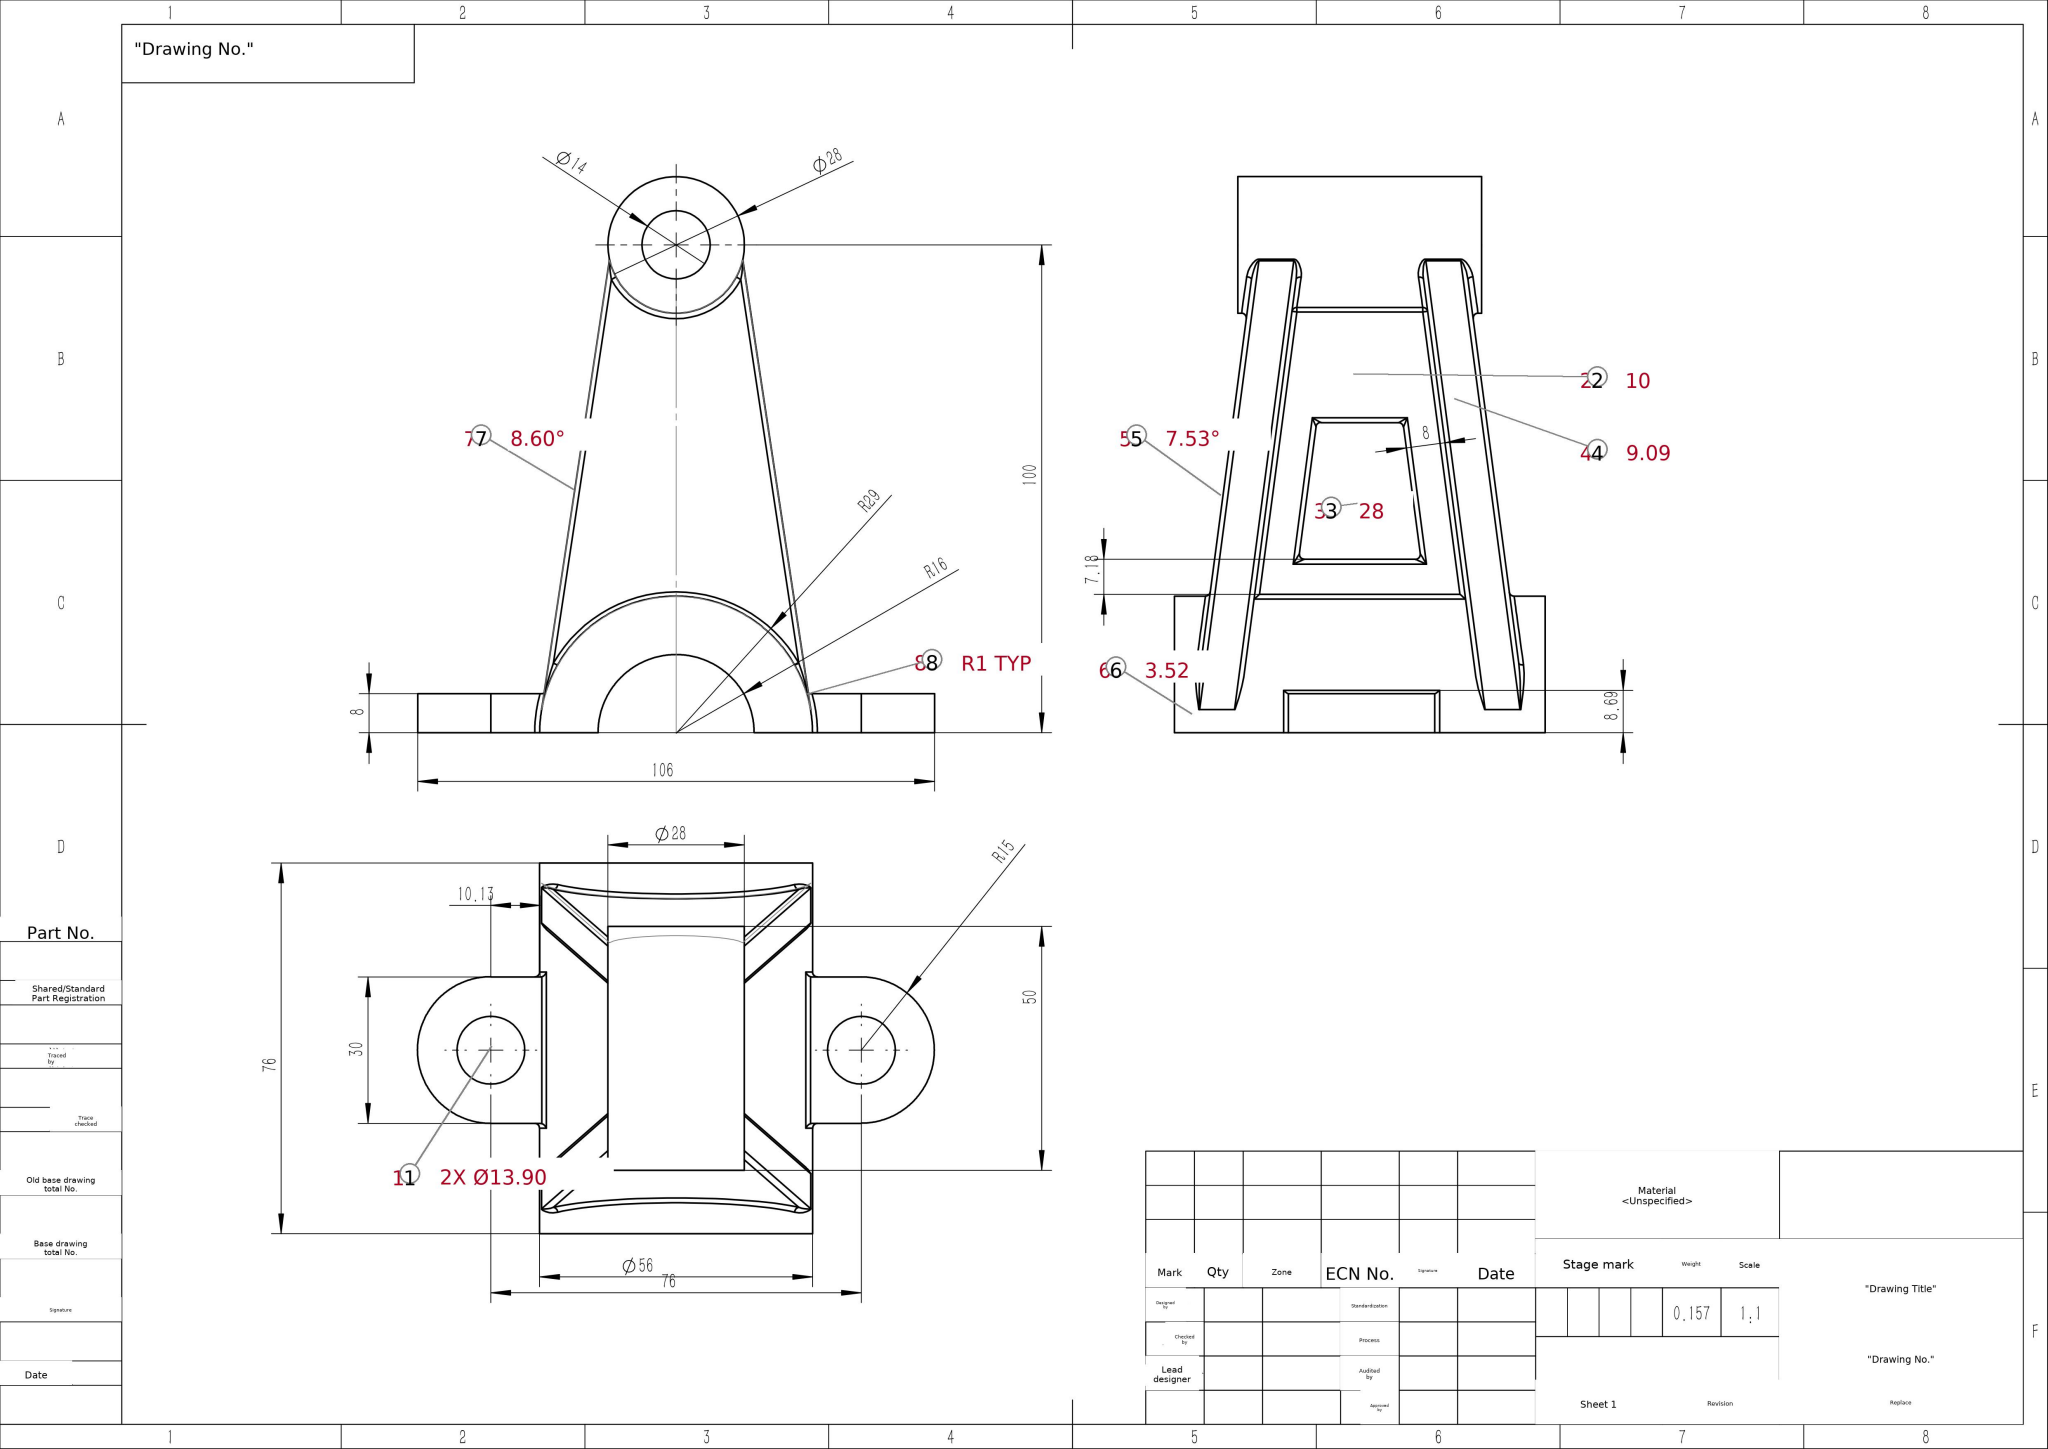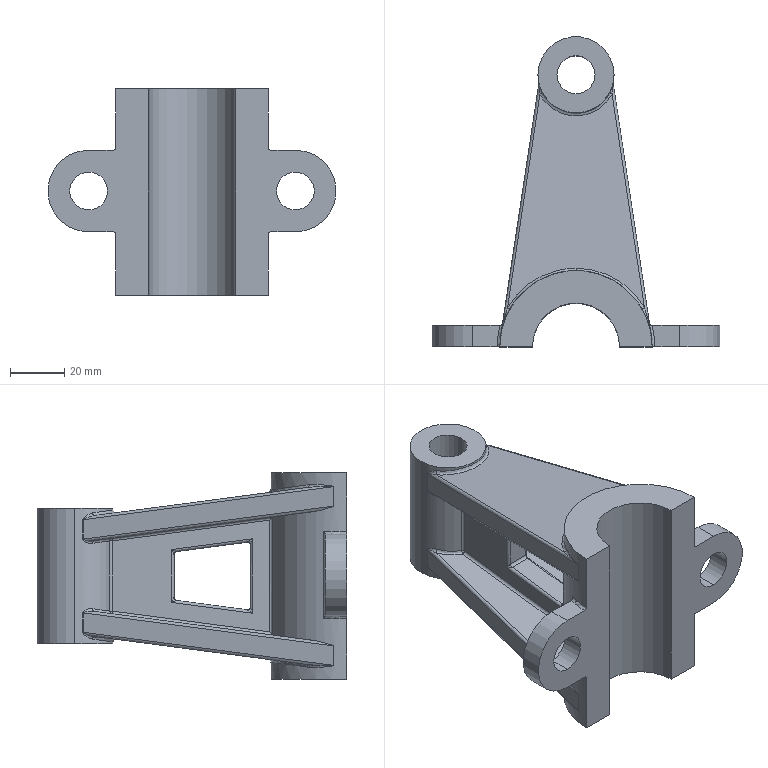Part | SolidWorks | mm | 1 solid | 119 faces | box 106 x 114 x 76 mm | volume 156955 mm3 | cylinder 49 | plane 32 | spline 30 | sphere 4 | torus 4 | commonest cylinder face diameters 2 x37 13.903 x4 14 x2 28 x2 30 x2 56 x1 32 x1